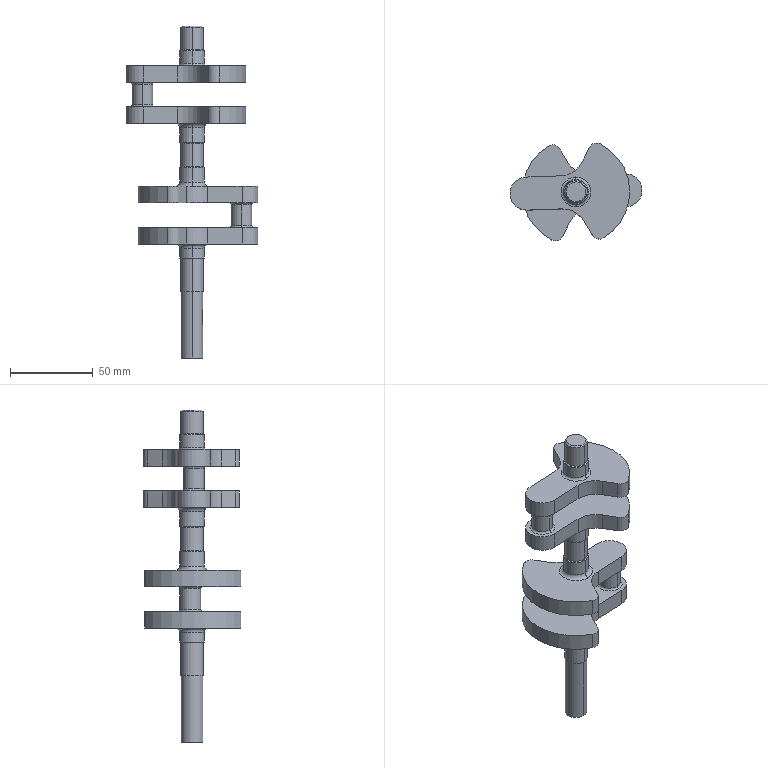Component | SolidWorks | MainCrankshaft-1 | 1 solid | 111 faces | box 79.96 x 59.05 x 201 mm | volume 110641 mm3 | cylinder 51 | plane 34 | torus 20 | cone 6 | commonest cylinder face diameters 10 x12 15 x8 30 x8 13.5 x6 12.5 x4 65 x4 20 x4 3 x3
build123d program:
from build123d import *

# Parameters (mm, degrees)
SKETCH1_R            = 30
BOSS_EXTRUDE1_DEPTH  = 90
SKETCH2_R            = 30
BOSS_EXTRUDE2_DEPTH  = 40
SKETCH3_R            = 25
BOSS_EXTRUDE3_DEPTH  = 60
BOSS_EXTRUDE4_DEPTH  = 40
SKETCH5_R            = 30
BOSS_EXTRUDE5_DEPTH  = 152
BOSS_EXTRUDE6_DEPTH  = 40
SKETCH7_R            = 25
BOSS_EXTRUDE7_DEPTH  = 60
BOSS_EXTRUDE8_DEPTH  = 40
SKETCH9_R            = 30
BOSS_EXTRUDE9_DEPTH  = 36
FILLET1_R            = 5
FILLET2_R            = 10
SKETCH10_R           = 30
BOSS_EXTRUDE10_DEPTH = 36
FILLET4_R            = 10
SKETCH11_R           = 27
BOSS_EXTRUDE11_DEPTH = 80
SKETCH12_OUTSIDE_W   = 375.636
SKETCH12_OUTSIDE_H   = 463.074
SKETCH12_OUTSIDE_R   = 27
CUT_EXTRUDE1_DEPTH   = 30
FILLET5_R            = 2
CHAMFER1_SIZE        = 2
FILLET6_R            = 6
SKETCH13_R           = 27
BOSS_EXTRUDE12_DEPTH = 60
CHAMFER2_SIZE        = 2
CHAMFER3_SIZE        = 3
SKETCH16_R           = 26
BOSS_EXTRUDE13_DEPTH = 160
CUT_EXTRUDE2_DEPTH   = 655.099
SCALE1_SCALE         = 0.25


with BuildPart() as part:
    # Sketch1 → Boss-Extrude1 (new body)
    with BuildSketch(Plane.XY):
        with Locations(Location((0, 0, 0), (0, 0, 180))):
            Circle(SKETCH1_R)
    extrude(amount=BOSS_EXTRUDE1_DEPTH)


with BuildPart() as body_2:
    # Sketch2 → Boss-Extrude2 (new body)
    # profile 1 of 2: a face of its own
    with BuildSketch(Plane.XY.offset(90)):
        with BuildLine():
            ThreePointArc((-113.786, -62.871), (0, -130), (113.786, -62.871))
            ThreePointArc((113.786, -62.871), (115.474, -47.575), (105.799, -35.609))
            Line((105.799, -35.609), (71.443, -17.016))
            ThreePointArc((71.443, -17.016), (48.457, 5.039), (40, 35.752))
            Line((40, 35.752), (40, 120))
            ThreePointArc((40, 120), (0, 160), (-40, 120))
            Line((-40, 120), (-40, 35.752))
            ThreePointArc((-40, 35.752), (-48.457, 5.039), (-71.443, -17.016))
            Line((-71.443, -17.016), (-105.799, -35.609))
            ThreePointArc((-105.799, -35.609), (-115.474, -47.575), (-113.786, -62.871))
        make_face()
        with Locations(Location((0, 0, 0), (0, 0, 180))):
            Circle(SKETCH2_R, mode=Mode.SUBTRACT)
    # profile 2 of 2: a face of its own
    with BuildSketch(Plane.XY.offset(90)):
        with Locations(Location((0, 0, 0), (0, 0, 180))):
            Circle(SKETCH2_R)
    extrude(amount=BOSS_EXTRUDE2_DEPTH)

    # Sketch3 → Boss-Extrude3 (add)
    with BuildSketch(Plane.XY.offset(130)):
        with Locations((0, 120)):
            Circle(SKETCH3_R)
    extrude(amount=BOSS_EXTRUDE3_DEPTH)

    # Sketch4 → Boss-Extrude4 (add)
    with BuildSketch(Plane.XY.offset(190)):
        with BuildLine():
            Line((105.799, -35.609), (71.443, -17.016))
            ThreePointArc((71.443, -17.016), (48.457, 5.039), (40, 35.752))
            Line((40, 35.752), (40, 120))
            ThreePointArc((40, 120), (0, 160), (-40, 120))
            Line((-40, 120), (-40, 35.752))
            ThreePointArc((-40, 35.752), (-48.457, 5.039), (-71.443, -17.016))
            Line((-71.443, -17.016), (-105.799, -35.609))
            ThreePointArc((-105.799, -35.609), (-115.474, -47.575), (-113.786, -62.871))
            ThreePointArc((-113.786, -62.871), (0, -130), (113.786, -62.871))
            ThreePointArc((113.786, -62.871), (115.474, -47.575), (105.799, -35.609))
        make_face()
    extrude(amount=BOSS_EXTRUDE4_DEPTH)

    # Sketch5 → Boss-Extrude5 (add)
    with BuildSketch(Plane.XY.offset(230)):
        Circle(SKETCH5_R)
    extrude(amount=BOSS_EXTRUDE5_DEPTH)

    # Sketch6 → Boss-Extrude6 (add)
    with BuildSketch(Plane.XY.offset(382)):
        with BuildLine():
            Line((40, -120), (40, -35.752))
            ThreePointArc((40, -35.752), (48.457, -5.039), (71.443, 17.016))
            Line((71.443, 17.016), (105.799, 35.609))
            ThreePointArc((105.799, 35.609), (115.474, 47.575), (113.786, 62.871))
            ThreePointArc((113.786, 62.871), (0, 130), (-113.786, 62.871))
            ThreePointArc((-113.786, 62.871), (-115.474, 47.575), (-105.799, 35.609))
            Line((-105.799, 35.609), (-71.443, 17.016))
            ThreePointArc((-71.443, 17.016), (-48.457, -5.039), (-40, -35.752))
            Line((-40, -35.752), (-40, -120))
            ThreePointArc((-40, -120), (0, -160), (40, -120))
        make_face()
    extrude(amount=BOSS_EXTRUDE6_DEPTH)

    # Sketch7 → Boss-Extrude7 (add)
    with BuildSketch(Plane.XY.offset(422)):
        with Locations((0, -120)):
            Circle(SKETCH7_R)
    extrude(amount=BOSS_EXTRUDE7_DEPTH)

    # Sketch8 → Boss-Extrude8 (add)
    with BuildSketch(Plane.XY.offset(482)):
        with BuildLine():
            Line((40, -120), (40, -35.752))
            ThreePointArc((40, -35.752), (48.457, -5.039), (71.443, 17.016))
            Line((71.443, 17.016), (105.799, 35.609))
            ThreePointArc((105.799, 35.609), (115.474, 47.575), (113.786, 62.871))
            ThreePointArc((113.786, 62.871), (0, 130), (-113.786, 62.871))
            ThreePointArc((-113.786, 62.871), (-115.474, 47.575), (-105.799, 35.609))
            Line((-105.799, 35.609), (-71.443, 17.016))
            ThreePointArc((-71.443, 17.016), (-48.457, -5.039), (-40, -35.752))
            Line((-40, -35.752), (-40, -120))
            ThreePointArc((-40, -120), (0, -160), (40, -120))
        make_face()
    extrude(amount=BOSS_EXTRUDE8_DEPTH)

    # Sketch9 → Boss-Extrude9 (add)
    with BuildSketch(Plane.XY.offset(522)):
        Circle(SKETCH9_R)
    extrude(amount=BOSS_EXTRUDE9_DEPTH)

    # Fillet1
    fillet1_edges = [body_2.edges().sort_by_distance(p)[0] for p in [
        (-25, 120, 130),
        (-25, 120, 190),
        (-25, -120, 422),
        (-25, -120, 482),
    ]]
    fillet(fillet1_edges, radius=FILLET1_R)

    # Fillet2
    fillet2_edges = [body_2.edges().sort_by_distance(p)[0] for p in [
        (-30, 0, 230),
        (-30, 0, 382),
    ]]
    fillet(fillet2_edges, radius=FILLET2_R)

    # Sketch10 → Boss-Extrude10 (add)
    with BuildSketch(Plane(origin=(0, 0, 90), x_dir=(-1, 0, 0), z_dir=(0, 0, -1))):
        with Locations(Location((0, 0, 0), (0, 0, 180))):
            Circle(SKETCH10_R)
    extrude(amount=BOSS_EXTRUDE10_DEPTH)

    # Fillet4
    fillet4_edges = [body_2.edges().sort_by_distance(p)[0] for p in [
        (-30, 0, 90),
    ]]
    fillet(fillet4_edges, radius=FILLET4_R)

    # Sketch11 → Boss-Extrude11 (add)
    with BuildSketch(Plane(origin=(0, 0, 54), x_dir=(-1, 0, 0), z_dir=(0, 0, -1))):
        Circle(SKETCH11_R)
    extrude(amount=BOSS_EXTRUDE11_DEPTH)

    # Sketch12 outside → Cut-Extrude1 (cut, symmetric)
    with BuildSketch(Plane(origin=(0, 0, 306), x_dir=(-1, 0, 0), z_dir=(0, 0, -1))):
        Rectangle(SKETCH12_OUTSIDE_W, SKETCH12_OUTSIDE_H)
        Circle(SKETCH12_OUTSIDE_R, mode=Mode.SUBTRACT)
    extrude(amount=CUT_EXTRUDE1_DEPTH, both=True, mode=Mode.SUBTRACT)

    # Fillet5
    fillet5_edges = [body_2.edges().sort_by_distance(p)[0] for p in [
        (27, 0, 336),
        (27, 0, 276),
    ]]
    fillet(fillet5_edges, radius=FILLET5_R)

    # Chamfer1
    chamfer1_edges = [body_2.edges().sort_by_distance(p)[0] for p in [
        (-30, 0, 54),
    ]]
    chamfer(chamfer1_edges, length=CHAMFER1_SIZE)

    # Fillet6
    fillet6_edges = [body_2.edges().sort_by_distance(p)[0] for p in [
        (-30, 0, 522),
    ]]
    fillet(fillet6_edges, radius=FILLET6_R)

    # Sketch13 → Boss-Extrude12 (add)
    with BuildSketch(Plane.XY.offset(558)):
        with Locations(Location((0, 0, 0), (0, 0, 180))):
            Circle(SKETCH13_R)
    extrude(amount=BOSS_EXTRUDE12_DEPTH)

    # Chamfer2
    chamfer2_edges = [body_2.edges().sort_by_distance(p)[0] for p in [
        (27, 0, 558),
    ]]
    chamfer(chamfer2_edges, length=CHAMFER2_SIZE)

    # Chamfer3
    chamfer3_edges = [body_2.edges().sort_by_distance(p)[0] for p in [
        (27, 0, 618),
    ]]
    chamfer(chamfer3_edges, length=CHAMFER3_SIZE)

    # Sketch16 → Boss-Extrude13 (add)
    with BuildSketch(Plane(origin=(0, 0, -26), x_dir=(-1, 0, 0), z_dir=(0, 0, -1))):
        Circle(SKETCH16_R)
    extrude(amount=BOSS_EXTRUDE13_DEPTH)

    # Sketch17 → Cut-Extrude2 (cut, through all)
    with BuildSketch(Plane(origin=(0, 20, 0), x_dir=(1, 0, 0), z_dir=(0, 1, 0))):
        with BuildLine():
            Line((6, 101), (6, 71))
            ThreePointArc((6, 71), (0, 65), (-6, 71))
            Line((-6, 71), (-6, 101))
            ThreePointArc((-6, 101), (0, 107), (6, 101))
        make_face()
    extrude(amount=CUT_EXTRUDE2_DEPTH, mode=Mode.SUBTRACT)


with BuildPart() as body_2_1:
    # Scale1: scaled about (2.94e-07, -0.008844, 284.204)
    add(body_2.part.scale(SCALE1_SCALE).moved(Location((0, -0.006633, 213.153))))


solid = body_2_1.part

# Placed as in the assembly
solid = solid.moved(Location((72.623, -251.6, -119.69), (0, 0, -87.981)))